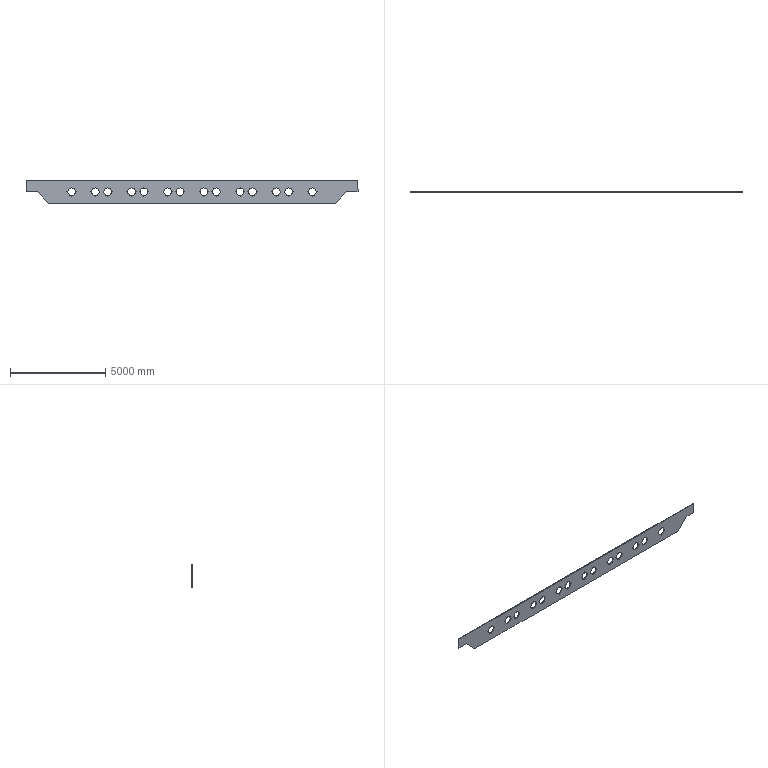Component | SolidWorks | ElectromagneticBeamWeb-1 | 1 solid | 150 faces | volume 723056342 mm3 | cylinder 140 | plane 10 | commonest cylinder face diameters 5 x112 400 x28 | material Plain Carbon Steel